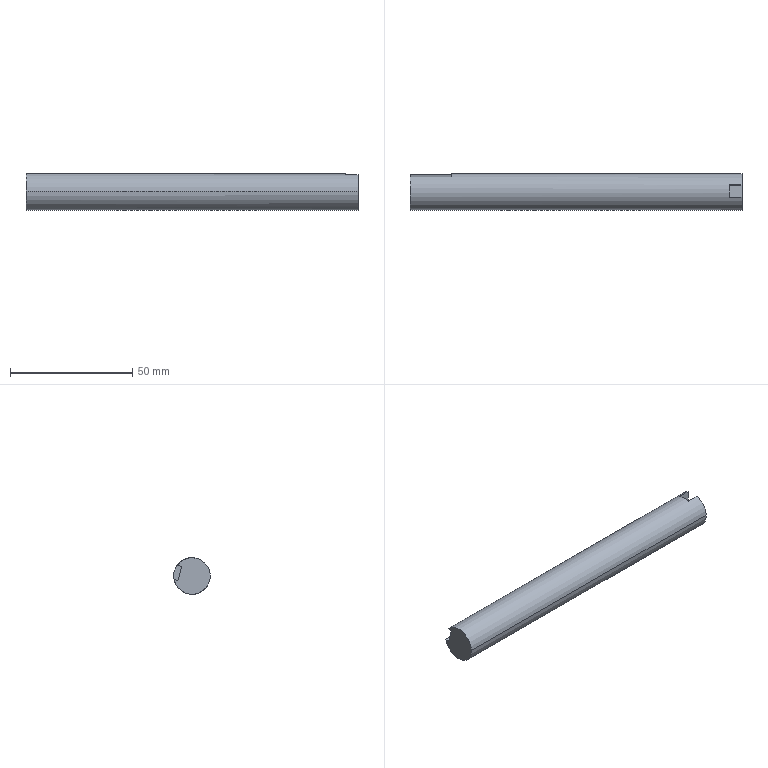Component | SolidWorks | GearAxis-1 | 1 solid | 12 faces | box 136 x 15 x 15 mm | volume 23676 mm3 | plane 10 | cylinder 2 | commonest cylinder face diameters 15 x2
build123d program:
from build123d import *

# Parameters (mm, degrees)
SKETCH2_R           = 7.5
BOSS_EXTRUDE1_DEPTH = 136
CUT_EXTRUDE1_START  = -17
CUT_EXTRUDE1_DEPTH  = 17
SKETCH4_W           = 5.222
SKETCH4_H           = 10.359
CUT_EXTRUDE2_DEPTH  = 5


with BuildPart() as part:
    # Sketch2 → Boss-Extrude1 (new body)
    with BuildSketch(Plane.XY):
        with Locations((0, 60.219)):
            Circle(SKETCH2_R)
    extrude(amount=-BOSS_EXTRUDE1_DEPTH)

    # Sketch3 → Cut-Extrude1 (cut)
    with BuildSketch(Plane.XY.offset(CUT_EXTRUDE1_START)):
        Polygon((-58.71, 75.553), (-10.152, 60.025), (-7.424, 59.153), (-5.833, 58.644), (-4.008, 64.351), (-5.833, 64.934), (-8.327, 65.732), (-56.885, 81.259), (-154.001, 112.314), (-155.826, 106.607), align=None)
    extrude(amount=CUT_EXTRUDE1_DEPTH, mode=Mode.SUBTRACT)

    # Sketch4 → Cut-Extrude2 (cut)
    with BuildSketch(Plane(origin=(0, 0, -136), x_dir=(-1, 0, 0), z_dir=(0, 0, -1))):
        with Locations((0, 67.719)):
            Rectangle(SKETCH4_W, SKETCH4_H)
    extrude(amount=-CUT_EXTRUDE2_DEPTH, mode=Mode.SUBTRACT)


solid = part.part

# Placed as in the assembly
solid = solid.moved(Location((-413, 57.007, -60.133), (86.943, -90, 0)))
STEP:
#1=COLOUR_RGB('',0.7922,0.8196,0.9333);
#2=FILL_AREA_STYLE_COLOUR('',#1);
#3=FILL_AREA_STYLE('',(#2));
#4=SURFACE_STYLE_FILL_AREA(#3);
#5=SURFACE_SIDE_STYLE('',(#4));
#6=SURFACE_STYLE_USAGE(.BOTH.,#5);
#7=PRESENTATION_STYLE_ASSIGNMENT((#6));
#8=CARTESIAN_POINT('',(-10.906,2.488,0.2709));
#9=VERTEX_POINT('',#8);
#10=CARTESIAN_POINT('',(-10.906,2.666,-0.01575));
#11=VERTEX_POINT('',#10);
#12=CARTESIAN_POINT('',(-10.906,2.371,-0.));
#13=DIRECTION('',(-1.,0.,-0.));
#14=DIRECTION('',(0.,-0.9986,0.05333));
#15=AXIS2_PLACEMENT_3D('',#12,#13,#14);
#16=CIRCLE('',#15,0.2953);
#17=EDGE_CURVE('',#9,#11,#16,.T.);
#18=ORIENTED_EDGE('',*,*,#17,.T.);
#19=CARTESIAN_POINT('',(-15.591,2.666,-0.01575));
#20=VERTEX_POINT('',#19);
#21=CARTESIAN_POINT('',(-10.906,2.666,-0.01575));
#22=DIRECTION('',(-1.,0.,-0.));
#23=VECTOR('',#22,39.37);
#24=LINE('',#21,#23);
#25=EDGE_CURVE('',#11,#20,#24,.T.);
#26=ORIENTED_EDGE('',*,*,#25,.T.);
#27=CARTESIAN_POINT('',(-15.591,2.61,0.1731));
#28=VERTEX_POINT('',#27);
#29=CARTESIAN_POINT('',(-15.591,2.371,-0.));
#30=DIRECTION('',(1.,-0.,0.));
#31=DIRECTION('',(0.,-0.9986,0.05333));
#32=AXIS2_PLACEMENT_3D('',#29,#30,#31);
#33=CIRCLE('',#32,0.2953);
#34=EDGE_CURVE('',#20,#28,#33,.T.);
#35=ORIENTED_EDGE('',*,*,#34,.T.);
#36=CARTESIAN_POINT('',(-16.26,2.61,0.1731));
#37=VERTEX_POINT('',#36);
#38=CARTESIAN_POINT('',(-15.307,2.61,0.1731));
#39=DIRECTION('',(-1.,0.,-0.));
#40=VECTOR('',#39,39.37);
#41=LINE('',#38,#40);
#42=EDGE_CURVE('',#28,#37,#41,.T.);
#43=ORIENTED_EDGE('',*,*,#42,.T.);
#44=CARTESIAN_POINT('',(-16.26,2.076,0.01575));
#45=VERTEX_POINT('',#44);
#46=CARTESIAN_POINT('',(-16.26,2.371,-0.));
#47=DIRECTION('',(-1.,0.,-0.));
#48=DIRECTION('',(0.,-0.9986,0.05333));
#49=AXIS2_PLACEMENT_3D('',#46,#47,#48);
#50=CIRCLE('',#49,0.2953);
#51=EDGE_CURVE('',#45,#37,#50,.T.);
#52=ORIENTED_EDGE('',*,*,#51,.F.);
#53=CARTESIAN_POINT('',(-10.906,2.076,0.01575));
#54=VERTEX_POINT('',#53);
#55=CARTESIAN_POINT('',(-10.906,2.076,0.01575));
#56=DIRECTION('',(-1.,0.,-0.));
#57=VECTOR('',#56,39.37);
#58=LINE('',#55,#57);
#59=EDGE_CURVE('',#54,#45,#58,.T.);
#60=ORIENTED_EDGE('',*,*,#59,.F.);
#61=CARTESIAN_POINT('',(-10.906,2.283,0.2819));
#62=VERTEX_POINT('',#61);
#63=CARTESIAN_POINT('',(-10.906,2.371,-0.));
#64=DIRECTION('',(-1.,0.,-0.));
#65=DIRECTION('',(0.,-0.9986,0.05333));
#66=AXIS2_PLACEMENT_3D('',#63,#64,#65);
#67=CIRCLE('',#66,0.2953);
#68=EDGE_CURVE('',#54,#62,#67,.T.);
#69=ORIENTED_EDGE('',*,*,#68,.T.);
#70=CARTESIAN_POINT('',(-11.102,2.283,0.2819));
#71=VERTEX_POINT('',#70);
#72=CARTESIAN_POINT('',(-10.906,2.283,0.2819));
#73=DIRECTION('',(1.,-0.,0.));
#74=VECTOR('',#73,39.37);
#75=LINE('',#72,#74);
#76=EDGE_CURVE('',#71,#62,#75,.T.);
#77=ORIENTED_EDGE('',*,*,#76,.F.);
#78=CARTESIAN_POINT('',(-11.102,2.488,0.2709));
#79=VERTEX_POINT('',#78);
#80=CARTESIAN_POINT('',(-11.102,2.371,-0.));
#81=DIRECTION('',(1.,-0.,0.));
#82=DIRECTION('',(0.,-0.9986,0.05333));
#83=AXIS2_PLACEMENT_3D('',#80,#81,#82);
#84=CIRCLE('',#83,0.2953);
#85=EDGE_CURVE('',#79,#71,#84,.T.);
#86=ORIENTED_EDGE('',*,*,#85,.F.);
#87=CARTESIAN_POINT('',(-10.906,2.488,0.2709));
#88=DIRECTION('',(-1.,0.,-0.));
#89=VECTOR('',#88,39.37);
#90=LINE('',#87,#89);
#91=EDGE_CURVE('',#9,#79,#90,.T.);
#92=ORIENTED_EDGE('',*,*,#91,.F.);
#93=EDGE_LOOP('',(#18,#26,#35,#43,#52,#60,#69,#77,#86,#92));
#94=FACE_OUTER_BOUND('',#93,.T.);
#95=CARTESIAN_POINT('',(-10.906,2.371,-0.));
#96=DIRECTION('',(-1.,0.,-0.));
#97=DIRECTION('',(0.,-0.9986,0.05333));
#98=AXIS2_PLACEMENT_3D('',#95,#96,#97);
#99=CYLINDRICAL_SURFACE('',#98,0.2953);
#100=ADVANCED_FACE('',(#94),#99,.T.);
#101=ORIENTED_EDGE('',*,*,#25,.F.);
#102=CARTESIAN_POINT('',(-10.906,2.371,-0.));
#103=DIRECTION('',(-1.,0.,-0.));
#104=DIRECTION('',(0.,-0.9986,0.05333));
#105=AXIS2_PLACEMENT_3D('',#102,#103,#104);
#106=CIRCLE('',#105,0.2953);
#107=EDGE_CURVE('',#11,#54,#106,.T.);
#108=ORIENTED_EDGE('',*,*,#107,.T.);
#109=ORIENTED_EDGE('',*,*,#59,.T.);
#110=CARTESIAN_POINT('',(-16.26,2.66,-0.0575));
#111=VERTEX_POINT('',#110);
#112=CARTESIAN_POINT('',(-16.26,2.371,-0.));
#113=DIRECTION('',(-1.,0.,-0.));
#114=DIRECTION('',(0.,-0.9986,0.05333));
#115=AXIS2_PLACEMENT_3D('',#112,#113,#114);
#116=CIRCLE('',#115,0.2953);
#117=EDGE_CURVE('',#111,#45,#116,.T.);
#118=ORIENTED_EDGE('',*,*,#117,.F.);
#119=CARTESIAN_POINT('',(-15.591,2.66,-0.0575));
#120=VERTEX_POINT('',#119);
#121=CARTESIAN_POINT('',(-15.307,2.66,-0.0575));
#122=DIRECTION('',(-1.,0.,-0.));
#123=VECTOR('',#122,39.37);
#124=LINE('',#121,#123);
#125=EDGE_CURVE('',#120,#111,#124,.T.);
#126=ORIENTED_EDGE('',*,*,#125,.F.);
#127=CARTESIAN_POINT('',(-15.591,2.371,-0.));
#128=DIRECTION('',(1.,-0.,0.));
#129=DIRECTION('',(0.,-0.9986,0.05333));
#130=AXIS2_PLACEMENT_3D('',#127,#128,#129);
#131=CIRCLE('',#130,0.2953);
#132=EDGE_CURVE('',#120,#20,#131,.T.);
#133=ORIENTED_EDGE('',*,*,#132,.T.);
#134=EDGE_LOOP('',(#101,#108,#109,#118,#126,#133));
#135=FACE_OUTER_BOUND('',#134,.T.);
#136=CARTESIAN_POINT('',(-10.906,2.371,-0.));
#137=DIRECTION('',(-1.,0.,-0.));
#138=DIRECTION('',(0.,-0.9986,0.05333));
#139=AXIS2_PLACEMENT_3D('',#136,#137,#138);
#140=CYLINDRICAL_SURFACE('',#139,0.2953);
#141=ADVANCED_FACE('',(#135),#140,.T.);
#142=ORIENTED_EDGE('',*,*,#117,.T.);
#143=ORIENTED_EDGE('',*,*,#51,.T.);
#144=CARTESIAN_POINT('',(-16.26,2.537,0.154));
#145=VERTEX_POINT('',#144);
#146=CARTESIAN_POINT('',(-16.26,1.645,-0.07955));
#147=DIRECTION('',(-0.,-0.9674,-0.2533));
#148=VECTOR('',#147,39.37);
#149=LINE('',#146,#148);
#150=EDGE_CURVE('',#37,#145,#149,.T.);
#151=ORIENTED_EDGE('',*,*,#150,.T.);
#152=CARTESIAN_POINT('',(-16.26,2.597,-0.07416));
#153=VERTEX_POINT('',#152);
#154=CARTESIAN_POINT('',(-16.26,3.136,-2.134));
#155=DIRECTION('',(-0.,-0.2533,0.9674));
#156=VECTOR('',#155,39.37);
#157=LINE('',#154,#156);
#158=EDGE_CURVE('',#153,#145,#157,.T.);
#159=ORIENTED_EDGE('',*,*,#158,.F.);
#160=CARTESIAN_POINT('',(-16.26,1.705,-0.3077));
#161=DIRECTION('',(-0.,-0.9674,-0.2533));
#162=VECTOR('',#161,39.37);
#163=LINE('',#160,#162);
#164=EDGE_CURVE('',#111,#153,#163,.T.);
#165=ORIENTED_EDGE('',*,*,#164,.F.);
#166=EDGE_LOOP('',(#142,#143,#151,#159,#165));
#167=FACE_OUTER_BOUND('',#166,.T.);
#168=CARTESIAN_POINT('',(-16.26,2.371,-0.));
#169=DIRECTION('',(-1.,0.,-0.));
#170=DIRECTION('',(-0.,-0.9986,0.05333));
#171=AXIS2_PLACEMENT_3D('',#168,#169,#170);
#172=PLANE('',#171);
#173=ADVANCED_FACE('',(#167),#172,.T.);
#174=ORIENTED_EDGE('',*,*,#17,.F.);
#175=CARTESIAN_POINT('',(-10.906,2.478,0.08575));
#176=VERTEX_POINT('',#175);
#177=CARTESIAN_POINT('',(-10.906,2.478,0.08575));
#178=DIRECTION('',(-0.,0.05333,0.9986));
#179=VECTOR('',#178,39.37);
#180=LINE('',#177,#179);
#181=EDGE_CURVE('',#176,#9,#180,.T.);
#182=ORIENTED_EDGE('',*,*,#181,.F.);
#183=CARTESIAN_POINT('',(-10.906,2.273,0.09671));
#184=VERTEX_POINT('',#183);
#185=CARTESIAN_POINT('',(-10.906,2.273,0.09671));
#186=DIRECTION('',(0.,0.9986,-0.05333));
#187=VECTOR('',#186,39.37);
#188=LINE('',#185,#187);
#189=EDGE_CURVE('',#184,#176,#188,.T.);
#190=ORIENTED_EDGE('',*,*,#189,.F.);
#191=CARTESIAN_POINT('',(-10.906,2.268,0.005482));
#192=DIRECTION('',(-0.,0.05333,0.9986));
#193=VECTOR('',#192,39.37);
#194=LINE('',#191,#193);
#195=EDGE_CURVE('',#184,#62,#194,.T.);
#196=ORIENTED_EDGE('',*,*,#195,.T.);
#197=ORIENTED_EDGE('',*,*,#68,.F.);
#198=ORIENTED_EDGE('',*,*,#107,.F.);
#199=EDGE_LOOP('',(#174,#182,#190,#196,#197,#198));
#200=FACE_OUTER_BOUND('',#199,.T.);
#201=CARTESIAN_POINT('',(-10.906,2.371,-0.));
#202=DIRECTION('',(-1.,0.,-0.));
#203=DIRECTION('',(-0.,-0.9986,0.05333));
#204=AXIS2_PLACEMENT_3D('',#201,#202,#203);
#205=PLANE('',#204);
#206=ADVANCED_FACE('',(#200),#205,.F.);
#207=CARTESIAN_POINT('',(-15.591,2.537,0.154));
#208=VERTEX_POINT('',#207);
#209=CARTESIAN_POINT('',(-15.307,2.537,0.154));
#210=DIRECTION('',(-1.,0.,-0.));
#211=VECTOR('',#210,39.37);
#212=LINE('',#209,#211);
#213=EDGE_CURVE('',#208,#145,#212,.T.);
#214=ORIENTED_EDGE('',*,*,#213,.T.);
#215=ORIENTED_EDGE('',*,*,#150,.F.);
#216=ORIENTED_EDGE('',*,*,#42,.F.);
#217=CARTESIAN_POINT('',(-15.591,1.645,-0.07955));
#218=DIRECTION('',(0.,0.9674,0.2533));
#219=VECTOR('',#218,39.37);
#220=LINE('',#217,#219);
#221=EDGE_CURVE('',#208,#28,#220,.T.);
#222=ORIENTED_EDGE('',*,*,#221,.F.);
#223=EDGE_LOOP('',(#214,#215,#216,#222));
#224=FACE_OUTER_BOUND('',#223,.T.);
#225=CARTESIAN_POINT('',(-15.307,1.645,-0.07955));
#226=DIRECTION('',(0.,0.2533,-0.9674));
#227=DIRECTION('',(-0.,-0.9674,-0.2533));
#228=AXIS2_PLACEMENT_3D('',#225,#226,#227);
#229=PLANE('',#228);
#230=ADVANCED_FACE('',(#224),#229,.T.);
#231=CARTESIAN_POINT('',(-15.591,2.597,-0.07416));
#232=VERTEX_POINT('',#231);
#233=CARTESIAN_POINT('',(-15.591,3.136,-2.134));
#234=DIRECTION('',(0.,0.2533,-0.9674));
#235=VECTOR('',#234,39.37);
#236=LINE('',#233,#235);
#237=EDGE_CURVE('',#208,#232,#236,.T.);
#238=ORIENTED_EDGE('',*,*,#237,.T.);
#239=CARTESIAN_POINT('',(-15.307,2.597,-0.07416));
#240=DIRECTION('',(-1.,0.,-0.));
#241=VECTOR('',#240,39.37);
#242=LINE('',#239,#241);
#243=EDGE_CURVE('',#232,#153,#242,.T.);
#244=ORIENTED_EDGE('',*,*,#243,.T.);
#245=ORIENTED_EDGE('',*,*,#158,.T.);
#246=ORIENTED_EDGE('',*,*,#213,.F.);
#247=EDGE_LOOP('',(#238,#244,#245,#246));
#248=FACE_OUTER_BOUND('',#247,.T.);
#249=CARTESIAN_POINT('',(-15.307,3.136,-2.134));
#250=DIRECTION('',(-0.,-0.9674,-0.2533));
#251=DIRECTION('',(-0.,-0.2533,0.9674));
#252=AXIS2_PLACEMENT_3D('',#249,#250,#251);
#253=PLANE('',#252);
#254=ADVANCED_FACE('',(#248),#253,.F.);
#255=CARTESIAN_POINT('',(-15.591,1.705,-0.3077));
#256=DIRECTION('',(0.,0.9674,0.2533));
#257=VECTOR('',#256,39.37);
#258=LINE('',#255,#257);
#259=EDGE_CURVE('',#232,#120,#258,.T.);
#260=ORIENTED_EDGE('',*,*,#259,.T.);
#261=ORIENTED_EDGE('',*,*,#125,.T.);
#262=ORIENTED_EDGE('',*,*,#164,.T.);
#263=ORIENTED_EDGE('',*,*,#243,.F.);
#264=EDGE_LOOP('',(#260,#261,#262,#263));
#265=FACE_OUTER_BOUND('',#264,.T.);
#266=CARTESIAN_POINT('',(-15.307,1.705,-0.3077));
#267=DIRECTION('',(0.,0.2533,-0.9674));
#268=DIRECTION('',(-0.,-0.9674,-0.2533));
#269=AXIS2_PLACEMENT_3D('',#266,#267,#268);
#270=PLANE('',#269);
#271=ADVANCED_FACE('',(#265),#270,.F.);
#272=ORIENTED_EDGE('',*,*,#237,.F.);
#273=ORIENTED_EDGE('',*,*,#221,.T.);
#274=ORIENTED_EDGE('',*,*,#34,.F.);
#275=ORIENTED_EDGE('',*,*,#132,.F.);
#276=ORIENTED_EDGE('',*,*,#259,.F.);
#277=EDGE_LOOP('',(#272,#273,#274,#275,#276));
#278=FACE_OUTER_BOUND('',#277,.T.);
#279=CARTESIAN_POINT('',(-15.591,2.371,-0.));
#280=DIRECTION('',(-1.,0.,-0.));
#281=DIRECTION('',(0.,0.9997,0.02574));
#282=AXIS2_PLACEMENT_3D('',#279,#280,#281);
#283=PLANE('',#282);
#284=ADVANCED_FACE('',(#278),#283,.T.);
#285=ORIENTED_EDGE('',*,*,#91,.T.);
#286=CARTESIAN_POINT('',(-11.102,2.478,0.08575));
#287=VERTEX_POINT('',#286);
#288=CARTESIAN_POINT('',(-11.102,2.478,0.08575));
#289=DIRECTION('',(-0.,0.05333,0.9986));
#290=VECTOR('',#289,39.37);
#291=LINE('',#288,#290);
#292=EDGE_CURVE('',#287,#79,#291,.T.);
#293=ORIENTED_EDGE('',*,*,#292,.F.);
#294=CARTESIAN_POINT('',(-11.102,2.478,0.08575));
#295=DIRECTION('',(1.,-0.,0.));
#296=VECTOR('',#295,39.37);
#297=LINE('',#294,#296);
#298=EDGE_CURVE('',#287,#176,#297,.T.);
#299=ORIENTED_EDGE('',*,*,#298,.T.);
#300=ORIENTED_EDGE('',*,*,#181,.T.);
#301=EDGE_LOOP('',(#285,#293,#299,#300));
#302=FACE_OUTER_BOUND('',#301,.T.);
#303=CARTESIAN_POINT('',(-11.102,2.478,0.08575));
#304=DIRECTION('',(0.,0.9986,-0.05333));
#305=DIRECTION('',(-1.,0.,-0.));
#306=AXIS2_PLACEMENT_3D('',#303,#304,#305);
#307=PLANE('',#306);
#308=ADVANCED_FACE('',(#302),#307,.F.);
#309=ORIENTED_EDGE('',*,*,#189,.T.);
#310=ORIENTED_EDGE('',*,*,#298,.F.);
#311=CARTESIAN_POINT('',(-11.102,2.273,0.09671));
#312=VERTEX_POINT('',#311);
#313=CARTESIAN_POINT('',(-11.102,2.273,0.09671));
#314=DIRECTION('',(0.,0.9986,-0.05333));
#315=VECTOR('',#314,39.37);
#316=LINE('',#313,#315);
#317=EDGE_CURVE('',#312,#287,#316,.T.);
#318=ORIENTED_EDGE('',*,*,#317,.F.);
#319=CARTESIAN_POINT('',(-11.102,2.273,0.09671));
#320=DIRECTION('',(1.,-0.,0.));
#321=VECTOR('',#320,39.37);
#322=LINE('',#319,#321);
#323=EDGE_CURVE('',#312,#184,#322,.T.);
#324=ORIENTED_EDGE('',*,*,#323,.T.);
#325=EDGE_LOOP('',(#309,#310,#318,#324));
#326=FACE_OUTER_BOUND('',#325,.T.);
#327=CARTESIAN_POINT('',(-11.102,2.273,0.09671));
#328=DIRECTION('',(0.,-0.05333,-0.9986));
#329=DIRECTION('',(1.,-0.,0.));
#330=AXIS2_PLACEMENT_3D('',#327,#328,#329);
#331=PLANE('',#330);
#332=ADVANCED_FACE('',(#326),#331,.F.);
#333=ORIENTED_EDGE('',*,*,#76,.T.);
#334=ORIENTED_EDGE('',*,*,#195,.F.);
#335=ORIENTED_EDGE('',*,*,#323,.F.);
#336=CARTESIAN_POINT('',(-11.102,2.273,0.09671));
#337=DIRECTION('',(0.,-0.05333,-0.9986));
#338=VECTOR('',#337,39.37);
#339=LINE('',#336,#338);
#340=EDGE_CURVE('',#71,#312,#339,.T.);
#341=ORIENTED_EDGE('',*,*,#340,.F.);
#342=EDGE_LOOP('',(#333,#334,#335,#341));
#343=FACE_OUTER_BOUND('',#342,.T.);
#344=CARTESIAN_POINT('',(-11.102,2.273,0.09671));
#345=DIRECTION('',(-0.,-0.9986,0.05333));
#346=DIRECTION('',(1.,-0.,0.));
#347=AXIS2_PLACEMENT_3D('',#344,#345,#346);
#348=PLANE('',#347);
#349=ADVANCED_FACE('',(#343),#348,.F.);
#350=ORIENTED_EDGE('',*,*,#85,.T.);
#351=ORIENTED_EDGE('',*,*,#340,.T.);
#352=ORIENTED_EDGE('',*,*,#317,.T.);
#353=ORIENTED_EDGE('',*,*,#292,.T.);
#354=EDGE_LOOP('',(#350,#351,#352,#353));
#355=FACE_OUTER_BOUND('',#354,.T.);
#356=CARTESIAN_POINT('',(-11.102,2.244,-2.367));
#357=DIRECTION('',(-1.,0.,-0.));
#358=DIRECTION('',(-0.,-0.9986,0.05333));
#359=AXIS2_PLACEMENT_3D('',#356,#357,#358);
#360=PLANE('',#359);
#361=ADVANCED_FACE('',(#355),#360,.F.);
#362=CLOSED_SHELL('',(#100,#141,#173,#206,#230,#254,#271,#284,#308,#332,#349,#361));
#363=MANIFOLD_SOLID_BREP('',#362);
#364=STYLED_ITEM('',(#7),#363);
#365=PRESENTATION_LAYER_ASSIGNMENT('','',(#364));
#366=CARTESIAN_POINT('',(0.,0.,0.));
#367=DIRECTION('',(0.,0.,1.));
#368=DIRECTION('',(1.,0.,0.));
#369=AXIS2_PLACEMENT_3D('',#366,#367,#368);
#370=(LENGTH_UNIT()NAMED_UNIT(*)SI_UNIT($,.METRE.));
#371=LENGTH_MEASURE_WITH_UNIT(LENGTH_MEASURE(0.0254),#370);
#372=DIMENSIONAL_EXPONENTS(1.,0.,0.,0.,0.,0.,0.);
#373=(CONVERSION_BASED_UNIT('',#371)LENGTH_UNIT()NAMED_UNIT(#372));
#374=UNCERTAINTY_MEASURE_WITH_UNIT(LENGTH_MEASURE(0.00001),#373,'','');
#375=(NAMED_UNIT(*)PLANE_ANGLE_UNIT()SI_UNIT($,.RADIAN.));
#376=(NAMED_UNIT(*)SI_UNIT($,.STERADIAN.)SOLID_ANGLE_UNIT());
#377=(GEOMETRIC_REPRESENTATION_CONTEXT(3)GLOBAL_UNCERTAINTY_ASSIGNED_CONTEXT((#374))GLOBAL_UNIT_ASSIGNED_CONTEXT((#373,#375,#376))REPRESENTATION_CONTEXT('',''));
#378=ADVANCED_BREP_SHAPE_REPRESENTATION('',(#363,#369),#377);
#379=(LENGTH_UNIT()NAMED_UNIT(*)SI_UNIT($,.METRE.));
#380=LENGTH_MEASURE_WITH_UNIT(LENGTH_MEASURE(0.0254),#379);
#381=DIMENSIONAL_EXPONENTS(1.,0.,0.,0.,0.,0.,0.);
#382=(CONVERSION_BASED_UNIT('',#380)LENGTH_UNIT()NAMED_UNIT(#381));
#383=UNCERTAINTY_MEASURE_WITH_UNIT(LENGTH_MEASURE(0.00001),#382,'','');
#384=(NAMED_UNIT(*)PLANE_ANGLE_UNIT()SI_UNIT($,.RADIAN.));
#385=(NAMED_UNIT(*)SI_UNIT($,.STERADIAN.)SOLID_ANGLE_UNIT());
#386=(GEOMETRIC_REPRESENTATION_CONTEXT(3)GLOBAL_UNCERTAINTY_ASSIGNED_CONTEXT((#383))GLOBAL_UNIT_ASSIGNED_CONTEXT((#382,#384,#385))REPRESENTATION_CONTEXT('',''));
#387=MECHANICAL_DESIGN_GEOMETRIC_PRESENTATION_REPRESENTATION('',(#364),#386);